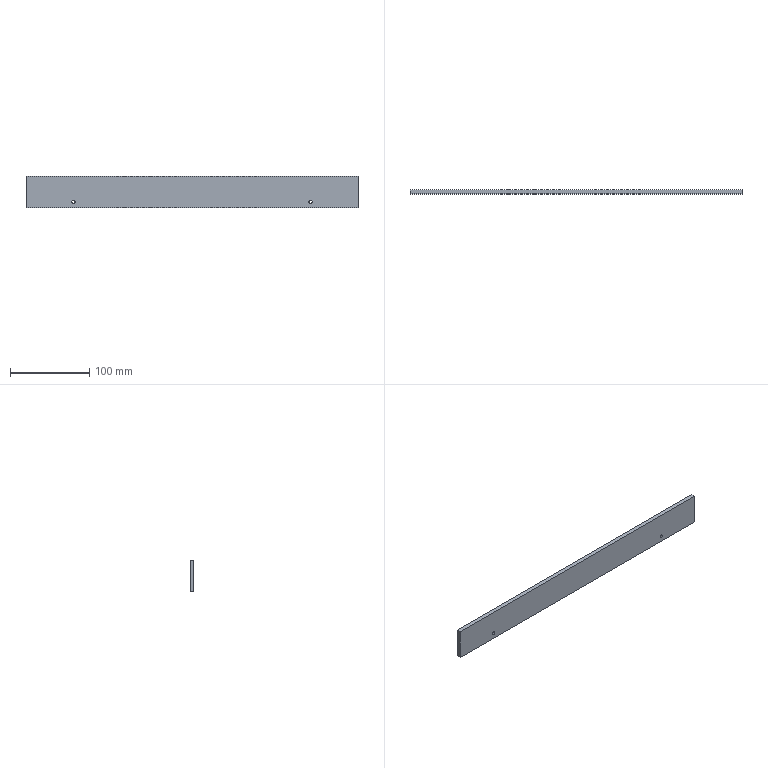Component | SolidWorks | BeefTendon-1 | 1 solid | 10 faces | box 420 x 5 x 40 mm | volume 83861 mm3 | plane 6 | cylinder 4 | commonest cylinder face diameters 4.2 x4
build123d program:
from build123d import *

# Parameters (mm, degrees)
SKETCH1_W                  = 420
SKETCH1_H                  = 40
BOSS_EXTRUDE1_DEPTH        = 5
F_4_2_4_2_DIAMETER_HOLE1_D = 4.2


with BuildPart() as part:
    # Sketch1 → Boss-Extrude1 (new body)
    with BuildSketch(Plane.XY):
        with Locations((210, 20)):
            Rectangle(SKETCH1_W, SKETCH1_H)
    extrude(amount=BOSS_EXTRUDE1_DEPTH)

    # 4.2 _4.2_ Diameter Hole1 (through all)
    with Locations(Plane(origin=(60, 32.5, 5), x_dir=(1, 0, 0), z_dir=(0, 0, 1))):
        with Locations((0, 0), (300, 0)):
            Hole(F_4_2_4_2_DIAMETER_HOLE1_D / 2)


solid = part.part

# Placed as in the assembly
solid = solid.moved(Location((-70, -221.728, 167.5), (-90, 0, 0)))
STEP:
#1=COLOUR_RGB('',0.7922,0.8196,0.9333);
#2=FILL_AREA_STYLE_COLOUR('',#1);
#3=FILL_AREA_STYLE('',(#2));
#4=SURFACE_STYLE_FILL_AREA(#3);
#5=SURFACE_SIDE_STYLE('',(#4));
#6=SURFACE_STYLE_USAGE(.BOTH.,#5);
#7=PRESENTATION_STYLE_ASSIGNMENT((#6));
#8=CARTESIAN_POINT('',(-0.4764,-8.729,5.315));
#9=VERTEX_POINT('',#8);
#10=CARTESIAN_POINT('',(-0.311,-8.729,5.315));
#11=VERTEX_POINT('',#10);
#12=CARTESIAN_POINT('',(-0.3937,-8.729,5.315));
#13=DIRECTION('',(-0.,1.,0.));
#14=DIRECTION('',(1.,0.,0.));
#15=AXIS2_PLACEMENT_3D('',#12,#13,#14);
#16=CIRCLE('',#15,0.08268);
#17=EDGE_CURVE('',#9,#11,#16,.T.);
#18=ORIENTED_EDGE('',*,*,#17,.F.);
#19=CARTESIAN_POINT('',(-0.4764,-8.533,5.315));
#20=VERTEX_POINT('',#19);
#21=CARTESIAN_POINT('',(-0.4764,-8.533,5.315));
#22=DIRECTION('',(-0.,1.,0.));
#23=VECTOR('',#22,39.37);
#24=LINE('',#21,#23);
#25=EDGE_CURVE('',#9,#20,#24,.T.);
#26=ORIENTED_EDGE('',*,*,#25,.T.);
#27=CARTESIAN_POINT('',(-0.311,-8.533,5.315));
#28=VERTEX_POINT('',#27);
#29=CARTESIAN_POINT('',(-0.3937,-8.533,5.315));
#30=DIRECTION('',(-0.,1.,0.));
#31=DIRECTION('',(1.,0.,0.));
#32=AXIS2_PLACEMENT_3D('',#29,#30,#31);
#33=CIRCLE('',#32,0.08268);
#34=EDGE_CURVE('',#20,#28,#33,.T.);
#35=ORIENTED_EDGE('',*,*,#34,.T.);
#36=CARTESIAN_POINT('',(-0.311,-8.533,5.315));
#37=DIRECTION('',(-0.,1.,0.));
#38=VECTOR('',#37,39.37);
#39=LINE('',#36,#38);
#40=EDGE_CURVE('',#11,#28,#39,.T.);
#41=ORIENTED_EDGE('',*,*,#40,.F.);
#42=EDGE_LOOP('',(#18,#26,#35,#41));
#43=FACE_OUTER_BOUND('',#42,.T.);
#44=CARTESIAN_POINT('',(-0.3937,-8.533,5.315));
#45=DIRECTION('',(-0.,1.,0.));
#46=DIRECTION('',(1.,0.,0.));
#47=AXIS2_PLACEMENT_3D('',#44,#45,#46);
#48=CYLINDRICAL_SURFACE('',#47,0.08268);
#49=ADVANCED_FACE('',(#43),#48,.F.);
#50=CARTESIAN_POINT('',(11.335,-8.729,5.315));
#51=VERTEX_POINT('',#50);
#52=CARTESIAN_POINT('',(11.5,-8.729,5.315));
#53=VERTEX_POINT('',#52);
#54=CARTESIAN_POINT('',(11.417,-8.729,5.315));
#55=DIRECTION('',(-0.,1.,0.));
#56=DIRECTION('',(1.,0.,0.));
#57=AXIS2_PLACEMENT_3D('',#54,#55,#56);
#58=CIRCLE('',#57,0.08268);
#59=EDGE_CURVE('',#51,#53,#58,.T.);
#60=ORIENTED_EDGE('',*,*,#59,.F.);
#61=CARTESIAN_POINT('',(11.335,-8.533,5.315));
#62=VERTEX_POINT('',#61);
#63=CARTESIAN_POINT('',(11.335,-8.533,5.315));
#64=DIRECTION('',(-0.,1.,0.));
#65=VECTOR('',#64,39.37);
#66=LINE('',#63,#65);
#67=EDGE_CURVE('',#51,#62,#66,.T.);
#68=ORIENTED_EDGE('',*,*,#67,.T.);
#69=CARTESIAN_POINT('',(11.5,-8.533,5.315));
#70=VERTEX_POINT('',#69);
#71=CARTESIAN_POINT('',(11.417,-8.533,5.315));
#72=DIRECTION('',(-0.,1.,0.));
#73=DIRECTION('',(1.,0.,0.));
#74=AXIS2_PLACEMENT_3D('',#71,#72,#73);
#75=CIRCLE('',#74,0.08268);
#76=EDGE_CURVE('',#62,#70,#75,.T.);
#77=ORIENTED_EDGE('',*,*,#76,.T.);
#78=CARTESIAN_POINT('',(11.5,-8.533,5.315));
#79=DIRECTION('',(-0.,1.,0.));
#80=VECTOR('',#79,39.37);
#81=LINE('',#78,#80);
#82=EDGE_CURVE('',#53,#70,#81,.T.);
#83=ORIENTED_EDGE('',*,*,#82,.F.);
#84=EDGE_LOOP('',(#60,#68,#77,#83));
#85=FACE_OUTER_BOUND('',#84,.T.);
#86=CARTESIAN_POINT('',(11.417,-8.533,5.315));
#87=DIRECTION('',(-0.,1.,0.));
#88=DIRECTION('',(1.,0.,0.));
#89=AXIS2_PLACEMENT_3D('',#86,#87,#88);
#90=CYLINDRICAL_SURFACE('',#89,0.08268);
#91=ADVANCED_FACE('',(#85),#90,.F.);
#92=CARTESIAN_POINT('',(-2.756,-8.729,5.02));
#93=VERTEX_POINT('',#92);
#94=CARTESIAN_POINT('',(-2.756,-8.729,6.594));
#95=VERTEX_POINT('',#94);
#96=CARTESIAN_POINT('',(-2.756,-8.729,6.594));
#97=DIRECTION('',(-0.,-0.,1.));
#98=VECTOR('',#97,39.37);
#99=LINE('',#96,#98);
#100=EDGE_CURVE('',#93,#95,#99,.T.);
#101=ORIENTED_EDGE('',*,*,#100,.T.);
#102=CARTESIAN_POINT('',(-2.756,-8.533,6.594));
#103=VERTEX_POINT('',#102);
#104=CARTESIAN_POINT('',(-2.756,-8.533,6.594));
#105=DIRECTION('',(0.,-1.,-0.));
#106=VECTOR('',#105,39.37);
#107=LINE('',#104,#106);
#108=EDGE_CURVE('',#103,#95,#107,.T.);
#109=ORIENTED_EDGE('',*,*,#108,.F.);
#110=CARTESIAN_POINT('',(-2.756,-8.533,5.02));
#111=VERTEX_POINT('',#110);
#112=CARTESIAN_POINT('',(-2.756,-8.533,6.594));
#113=DIRECTION('',(-0.,-0.,1.));
#114=VECTOR('',#113,39.37);
#115=LINE('',#112,#114);
#116=EDGE_CURVE('',#111,#103,#115,.T.);
#117=ORIENTED_EDGE('',*,*,#116,.F.);
#118=CARTESIAN_POINT('',(-2.756,-8.533,5.02));
#119=DIRECTION('',(0.,-1.,-0.));
#120=VECTOR('',#119,39.37);
#121=LINE('',#118,#120);
#122=EDGE_CURVE('',#111,#93,#121,.T.);
#123=ORIENTED_EDGE('',*,*,#122,.T.);
#124=EDGE_LOOP('',(#101,#109,#117,#123));
#125=FACE_OUTER_BOUND('',#124,.T.);
#126=CARTESIAN_POINT('',(-2.756,-8.533,6.594));
#127=DIRECTION('',(1.,0.,0.));
#128=DIRECTION('',(0.,-1.,-0.));
#129=AXIS2_PLACEMENT_3D('',#126,#127,#128);
#130=PLANE('',#129);
#131=ADVANCED_FACE('',(#125),#130,.F.);
#132=CARTESIAN_POINT('',(13.78,-8.729,6.594));
#133=VERTEX_POINT('',#132);
#134=CARTESIAN_POINT('',(-2.756,-8.729,6.594));
#135=DIRECTION('',(1.,0.,0.));
#136=VECTOR('',#135,39.37);
#137=LINE('',#134,#136);
#138=EDGE_CURVE('',#95,#133,#137,.T.);
#139=ORIENTED_EDGE('',*,*,#138,.T.);
#140=CARTESIAN_POINT('',(13.78,-8.533,6.594));
#141=VERTEX_POINT('',#140);
#142=CARTESIAN_POINT('',(13.78,-8.533,6.594));
#143=DIRECTION('',(0.,-1.,-0.));
#144=VECTOR('',#143,39.37);
#145=LINE('',#142,#144);
#146=EDGE_CURVE('',#141,#133,#145,.T.);
#147=ORIENTED_EDGE('',*,*,#146,.F.);
#148=CARTESIAN_POINT('',(-2.756,-8.533,6.594));
#149=DIRECTION('',(1.,0.,0.));
#150=VECTOR('',#149,39.37);
#151=LINE('',#148,#150);
#152=EDGE_CURVE('',#103,#141,#151,.T.);
#153=ORIENTED_EDGE('',*,*,#152,.F.);
#154=ORIENTED_EDGE('',*,*,#108,.T.);
#155=EDGE_LOOP('',(#139,#147,#153,#154));
#156=FACE_OUTER_BOUND('',#155,.T.);
#157=CARTESIAN_POINT('',(-2.756,-8.533,6.594));
#158=DIRECTION('',(0.,0.,-1.));
#159=DIRECTION('',(-0.,1.,0.));
#160=AXIS2_PLACEMENT_3D('',#157,#158,#159);
#161=PLANE('',#160);
#162=ADVANCED_FACE('',(#156),#161,.F.);
#163=CARTESIAN_POINT('',(13.78,-8.729,5.02));
#164=VERTEX_POINT('',#163);
#165=CARTESIAN_POINT('',(13.78,-8.729,6.594));
#166=DIRECTION('',(0.,0.,-1.));
#167=VECTOR('',#166,39.37);
#168=LINE('',#165,#167);
#169=EDGE_CURVE('',#133,#164,#168,.T.);
#170=ORIENTED_EDGE('',*,*,#169,.T.);
#171=CARTESIAN_POINT('',(13.78,-8.533,5.02));
#172=VERTEX_POINT('',#171);
#173=CARTESIAN_POINT('',(13.78,-8.533,5.02));
#174=DIRECTION('',(0.,-1.,-0.));
#175=VECTOR('',#174,39.37);
#176=LINE('',#173,#175);
#177=EDGE_CURVE('',#172,#164,#176,.T.);
#178=ORIENTED_EDGE('',*,*,#177,.F.);
#179=CARTESIAN_POINT('',(13.78,-8.533,6.594));
#180=DIRECTION('',(0.,0.,-1.));
#181=VECTOR('',#180,39.37);
#182=LINE('',#179,#181);
#183=EDGE_CURVE('',#141,#172,#182,.T.);
#184=ORIENTED_EDGE('',*,*,#183,.F.);
#185=ORIENTED_EDGE('',*,*,#146,.T.);
#186=EDGE_LOOP('',(#170,#178,#184,#185));
#187=FACE_OUTER_BOUND('',#186,.T.);
#188=CARTESIAN_POINT('',(13.78,-8.533,6.594));
#189=DIRECTION('',(-1.,-0.,-0.));
#190=DIRECTION('',(-0.,1.,0.));
#191=AXIS2_PLACEMENT_3D('',#188,#189,#190);
#192=PLANE('',#191);
#193=ADVANCED_FACE('',(#187),#192,.F.);
#194=CARTESIAN_POINT('',(-2.756,-8.729,5.02));
#195=DIRECTION('',(-1.,-0.,-0.));
#196=VECTOR('',#195,39.37);
#197=LINE('',#194,#196);
#198=EDGE_CURVE('',#164,#93,#197,.T.);
#199=ORIENTED_EDGE('',*,*,#198,.T.);
#200=ORIENTED_EDGE('',*,*,#122,.F.);
#201=CARTESIAN_POINT('',(-2.756,-8.533,5.02));
#202=DIRECTION('',(-1.,-0.,-0.));
#203=VECTOR('',#202,39.37);
#204=LINE('',#201,#203);
#205=EDGE_CURVE('',#172,#111,#204,.T.);
#206=ORIENTED_EDGE('',*,*,#205,.F.);
#207=ORIENTED_EDGE('',*,*,#177,.T.);
#208=EDGE_LOOP('',(#199,#200,#206,#207));
#209=FACE_OUTER_BOUND('',#208,.T.);
#210=CARTESIAN_POINT('',(-2.756,-8.533,5.02));
#211=DIRECTION('',(-0.,-0.,1.));
#212=DIRECTION('',(0.,-1.,-0.));
#213=AXIS2_PLACEMENT_3D('',#210,#211,#212);
#214=PLANE('',#213);
#215=ADVANCED_FACE('',(#209),#214,.F.);
#216=CARTESIAN_POINT('',(-0.3937,-8.533,5.315));
#217=DIRECTION('',(-0.,1.,0.));
#218=DIRECTION('',(1.,0.,0.));
#219=AXIS2_PLACEMENT_3D('',#216,#217,#218);
#220=CIRCLE('',#219,0.08268);
#221=EDGE_CURVE('',#28,#20,#220,.T.);
#222=ORIENTED_EDGE('',*,*,#221,.F.);
#223=ORIENTED_EDGE('',*,*,#34,.F.);
#224=EDGE_LOOP('',(#222,#223));
#225=FACE_BOUND('',#224,.T.);
#226=CARTESIAN_POINT('',(11.417,-8.533,5.315));
#227=DIRECTION('',(-0.,1.,0.));
#228=DIRECTION('',(1.,0.,0.));
#229=AXIS2_PLACEMENT_3D('',#226,#227,#228);
#230=CIRCLE('',#229,0.08268);
#231=EDGE_CURVE('',#70,#62,#230,.T.);
#232=ORIENTED_EDGE('',*,*,#231,.F.);
#233=ORIENTED_EDGE('',*,*,#76,.F.);
#234=EDGE_LOOP('',(#232,#233));
#235=FACE_BOUND('',#234,.T.);
#236=ORIENTED_EDGE('',*,*,#116,.T.);
#237=ORIENTED_EDGE('',*,*,#152,.T.);
#238=ORIENTED_EDGE('',*,*,#183,.T.);
#239=ORIENTED_EDGE('',*,*,#205,.T.);
#240=EDGE_LOOP('',(#236,#237,#238,#239));
#241=FACE_OUTER_BOUND('',#240,.T.);
#242=CARTESIAN_POINT('',(-2.756,-8.533,6.594));
#243=DIRECTION('',(0.,-1.,-0.));
#244=DIRECTION('',(-1.,-0.,-0.));
#245=AXIS2_PLACEMENT_3D('',#242,#243,#244);
#246=PLANE('',#245);
#247=ADVANCED_FACE('',(#225,#235,#241),#246,.F.);
#248=CARTESIAN_POINT('',(-0.3937,-8.729,5.315));
#249=DIRECTION('',(-0.,1.,0.));
#250=DIRECTION('',(1.,0.,0.));
#251=AXIS2_PLACEMENT_3D('',#248,#249,#250);
#252=CIRCLE('',#251,0.08268);
#253=EDGE_CURVE('',#11,#9,#252,.T.);
#254=ORIENTED_EDGE('',*,*,#253,.T.);
#255=ORIENTED_EDGE('',*,*,#17,.T.);
#256=EDGE_LOOP('',(#254,#255));
#257=FACE_BOUND('',#256,.T.);
#258=CARTESIAN_POINT('',(11.417,-8.729,5.315));
#259=DIRECTION('',(-0.,1.,0.));
#260=DIRECTION('',(1.,0.,0.));
#261=AXIS2_PLACEMENT_3D('',#258,#259,#260);
#262=CIRCLE('',#261,0.08268);
#263=EDGE_CURVE('',#53,#51,#262,.T.);
#264=ORIENTED_EDGE('',*,*,#263,.T.);
#265=ORIENTED_EDGE('',*,*,#59,.T.);
#266=EDGE_LOOP('',(#264,#265));
#267=FACE_BOUND('',#266,.T.);
#268=ORIENTED_EDGE('',*,*,#100,.F.);
#269=ORIENTED_EDGE('',*,*,#198,.F.);
#270=ORIENTED_EDGE('',*,*,#169,.F.);
#271=ORIENTED_EDGE('',*,*,#138,.F.);
#272=EDGE_LOOP('',(#268,#269,#270,#271));
#273=FACE_OUTER_BOUND('',#272,.T.);
#274=CARTESIAN_POINT('',(-2.756,-8.729,6.594));
#275=DIRECTION('',(0.,-1.,-0.));
#276=DIRECTION('',(-1.,-0.,-0.));
#277=AXIS2_PLACEMENT_3D('',#274,#275,#276);
#278=PLANE('',#277);
#279=ADVANCED_FACE('',(#257,#267,#273),#278,.T.);
#280=ORIENTED_EDGE('',*,*,#67,.F.);
#281=ORIENTED_EDGE('',*,*,#263,.F.);
#282=ORIENTED_EDGE('',*,*,#82,.T.);
#283=ORIENTED_EDGE('',*,*,#231,.T.);
#284=EDGE_LOOP('',(#280,#281,#282,#283));
#285=FACE_OUTER_BOUND('',#284,.T.);
#286=CARTESIAN_POINT('',(11.417,-8.533,5.315));
#287=DIRECTION('',(-0.,1.,0.));
#288=DIRECTION('',(1.,0.,0.));
#289=AXIS2_PLACEMENT_3D('',#286,#287,#288);
#290=CYLINDRICAL_SURFACE('',#289,0.08268);
#291=ADVANCED_FACE('',(#285),#290,.F.);
#292=ORIENTED_EDGE('',*,*,#25,.F.);
#293=ORIENTED_EDGE('',*,*,#253,.F.);
#294=ORIENTED_EDGE('',*,*,#40,.T.);
#295=ORIENTED_EDGE('',*,*,#221,.T.);
#296=EDGE_LOOP('',(#292,#293,#294,#295));
#297=FACE_OUTER_BOUND('',#296,.T.);
#298=CARTESIAN_POINT('',(-0.3937,-8.533,5.315));
#299=DIRECTION('',(-0.,1.,0.));
#300=DIRECTION('',(1.,0.,0.));
#301=AXIS2_PLACEMENT_3D('',#298,#299,#300);
#302=CYLINDRICAL_SURFACE('',#301,0.08268);
#303=ADVANCED_FACE('',(#297),#302,.F.);
#304=CLOSED_SHELL('',(#49,#91,#131,#162,#193,#215,#247,#279,#291,#303));
#305=MANIFOLD_SOLID_BREP('',#304);
#306=STYLED_ITEM('',(#7),#305);
#307=PRESENTATION_LAYER_ASSIGNMENT('','',(#306));
#308=(LENGTH_UNIT()NAMED_UNIT(*)SI_UNIT($,.METRE.));
#309=LENGTH_MEASURE_WITH_UNIT(LENGTH_MEASURE(0.0254),#308);
#310=DIMENSIONAL_EXPONENTS(1.,0.,0.,0.,0.,0.,0.);
#311=(CONVERSION_BASED_UNIT('',#309)LENGTH_UNIT()NAMED_UNIT(#310));
#312=UNCERTAINTY_MEASURE_WITH_UNIT(LENGTH_MEASURE(0.00001),#311,'','');
#313=(NAMED_UNIT(*)PLANE_ANGLE_UNIT()SI_UNIT($,.RADIAN.));
#314=(NAMED_UNIT(*)SI_UNIT($,.STERADIAN.)SOLID_ANGLE_UNIT());
#315=(GEOMETRIC_REPRESENTATION_CONTEXT(3)GLOBAL_UNCERTAINTY_ASSIGNED_CONTEXT((#312))GLOBAL_UNIT_ASSIGNED_CONTEXT((#311,#313,#314))REPRESENTATION_CONTEXT('',''));
#316=MECHANICAL_DESIGN_GEOMETRIC_PRESENTATION_REPRESENTATION('',(#306),#315);
#317=CARTESIAN_POINT('',(0.,0.,0.));
#318=DIRECTION('',(0.,0.,1.));
#319=DIRECTION('',(1.,0.,0.));
#320=AXIS2_PLACEMENT_3D('',#317,#318,#319);
#321=(LENGTH_UNIT()NAMED_UNIT(*)SI_UNIT($,.METRE.));
#322=LENGTH_MEASURE_WITH_UNIT(LENGTH_MEASURE(0.0254),#321);
#323=DIMENSIONAL_EXPONENTS(1.,0.,0.,0.,0.,0.,0.);
#324=(CONVERSION_BASED_UNIT('',#322)LENGTH_UNIT()NAMED_UNIT(#323));
#325=UNCERTAINTY_MEASURE_WITH_UNIT(LENGTH_MEASURE(0.00001),#324,'','');
#326=(NAMED_UNIT(*)PLANE_ANGLE_UNIT()SI_UNIT($,.RADIAN.));
#327=(NAMED_UNIT(*)SI_UNIT($,.STERADIAN.)SOLID_ANGLE_UNIT());
#328=(GEOMETRIC_REPRESENTATION_CONTEXT(3)GLOBAL_UNCERTAINTY_ASSIGNED_CONTEXT((#325))GLOBAL_UNIT_ASSIGNED_CONTEXT((#324,#326,#327))REPRESENTATION_CONTEXT('',''));
#329=ADVANCED_BREP_SHAPE_REPRESENTATION('',(#305,#320),#328);